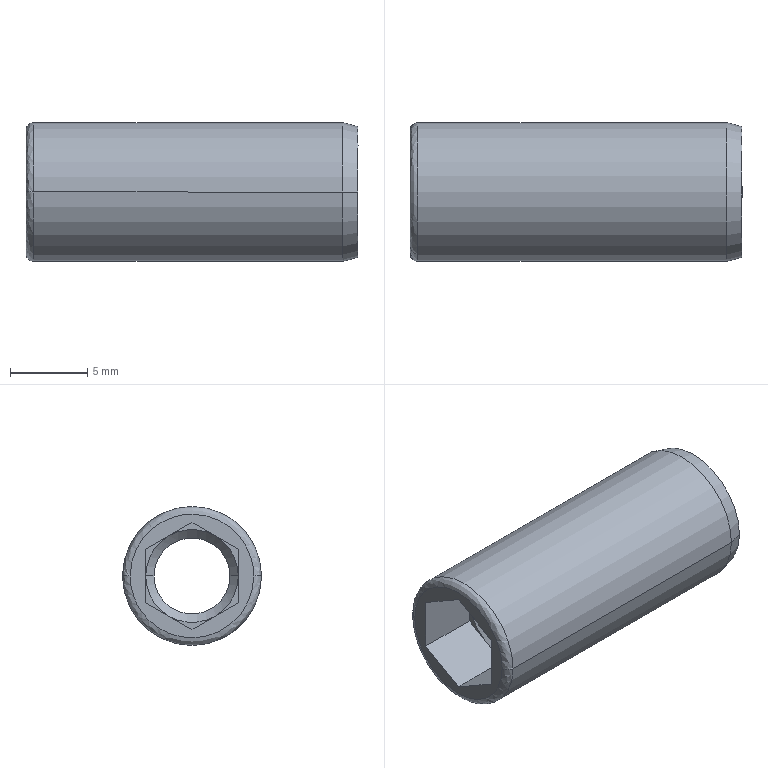Component | SolidWorks | HZ022-SC32x100S-1_HZ022-SC32x100S (10)-1 | 1 solid | 27 faces | box 21.5 x 9 x 9 mm | volume 818 mm3 | plane 15 | cylinder 6 | cone 4 | spline 2 | commonest cylinder face diameters 6.02 x2 9 x2 4.917 x2 | material AL6061
STEP:
#1=CARTESIAN_POINT('',(-11.105,4.179,35.846));
#2=VERTEX_POINT('',#1);
#3=CARTESIAN_POINT('',(-11.105,4.494,35.846));
#4=VERTEX_POINT('',#3);
#5=CARTESIAN_POINT('',(-11.105,4.179,35.846));
#6=CARTESIAN_POINT('',(-11.105,4.179,35.531));
#7=CARTESIAN_POINT('',(-11.105,4.494,35.531));
#8=CARTESIAN_POINT('',(-11.105,4.494,35.846));
#9=(BOUNDED_CURVE()B_SPLINE_CURVE(3,(#5,#6,#7,#8),.UNSPECIFIED.,.F.,.T.)B_SPLINE_CURVE_WITH_KNOTS((4,4),(0.,1.),.UNSPECIFIED.)CURVE()GEOMETRIC_REPRESENTATION_ITEM()RATIONAL_B_SPLINE_CURVE((1.,0.3333,0.3333,1.))REPRESENTATION_ITEM(''));
#10=EDGE_CURVE('',#2,#4,#9,.T.);
#11=ORIENTED_EDGE('',*,*,#10,.T.);
#12=CARTESIAN_POINT('',(-11.085,4.514,35.846));
#13=VERTEX_POINT('',#12);
#14=CARTESIAN_POINT('',(-11.085,4.494,35.846));
#15=DIRECTION('',(-0.,0.,-1.));
#16=DIRECTION('',(0.,1.,0.));
#17=AXIS2_PLACEMENT_3D('',#14,#15,#16);
#18=CIRCLE('',#17,0.01969);
#19=EDGE_CURVE('',#4,#13,#18,.T.);
#20=ORIENTED_EDGE('',*,*,#19,.T.);
#21=CARTESIAN_POINT('',(-11.085,4.16,35.846));
#22=VERTEX_POINT('',#21);
#23=CARTESIAN_POINT('',(-11.085,4.337,35.846));
#24=DIRECTION('',(1.,0.,-0.));
#25=DIRECTION('',(0.,-1.,0.));
#26=AXIS2_PLACEMENT_3D('',#23,#24,#25);
#27=CIRCLE('',#26,0.1772);
#28=EDGE_CURVE('',#22,#13,#27,.T.);
#29=ORIENTED_EDGE('',*,*,#28,.F.);
#30=CARTESIAN_POINT('',(-11.085,4.179,35.846));
#31=DIRECTION('',(0.,-0.,1.));
#32=DIRECTION('',(0.,-1.,0.));
#33=AXIS2_PLACEMENT_3D('',#30,#31,#32);
#34=CIRCLE('',#33,0.01969);
#35=EDGE_CURVE('',#2,#22,#34,.T.);
#36=ORIENTED_EDGE('',*,*,#35,.F.);
#37=EDGE_LOOP('',(#11,#20,#29,#36));
#38=FACE_OUTER_BOUND('',#37,.T.);
#39=CARTESIAN_POINT('',(-11.105,4.494,35.846));
#40=CARTESIAN_POINT('',(-11.105,4.494,35.531));
#41=CARTESIAN_POINT('',(-11.105,4.179,35.531));
#42=CARTESIAN_POINT('',(-11.105,4.179,35.846));
#43=CARTESIAN_POINT('',(-11.105,4.506,35.846));
#44=CARTESIAN_POINT('',(-11.105,4.506,35.508));
#45=CARTESIAN_POINT('',(-11.105,4.168,35.508));
#46=CARTESIAN_POINT('',(-11.105,4.168,35.846));
#47=CARTESIAN_POINT('',(-11.096,4.514,35.846));
#48=CARTESIAN_POINT('',(-11.096,4.514,35.492));
#49=CARTESIAN_POINT('',(-11.096,4.16,35.492));
#50=CARTESIAN_POINT('',(-11.096,4.16,35.846));
#51=CARTESIAN_POINT('',(-11.085,4.514,35.846));
#52=CARTESIAN_POINT('',(-11.085,4.514,35.492));
#53=CARTESIAN_POINT('',(-11.085,4.16,35.492));
#54=CARTESIAN_POINT('',(-11.085,4.16,35.846));
#55=(BOUNDED_SURFACE()B_SPLINE_SURFACE(3,3,((#39,#40,#41,#42),(#43,#44,#45,#46),(#47,#48,#49,#50),(#51,#52,#53,#54)),.UNSPECIFIED.,.F.,.F.,.F.)B_SPLINE_SURFACE_WITH_KNOTS((4,4),(4,4),(0.,1.),(0.,1.),.UNSPECIFIED.)GEOMETRIC_REPRESENTATION_ITEM()RATIONAL_B_SPLINE_SURFACE(((1.,0.3333,0.3333,1.),(0.8047,0.2682,0.2682,0.8047),(0.8047,0.2682,0.2682,0.8047),(1.,0.3333,0.3333,1.)))REPRESENTATION_ITEM('')SURFACE());
#56=ADVANCED_FACE('',(#38),#55,.T.);
#57=CARTESIAN_POINT('',(-10.258,4.218,35.846));
#58=VERTEX_POINT('',#57);
#59=CARTESIAN_POINT('',(-10.258,4.455,35.846));
#60=VERTEX_POINT('',#59);
#61=CARTESIAN_POINT('',(-10.258,4.337,35.846));
#62=DIRECTION('',(-1.,-0.,0.));
#63=DIRECTION('',(0.,-1.,0.));
#64=AXIS2_PLACEMENT_3D('',#61,#62,#63);
#65=CIRCLE('',#64,0.1185);
#66=EDGE_CURVE('',#58,#60,#65,.T.);
#67=ORIENTED_EDGE('',*,*,#66,.F.);
#68=CARTESIAN_POINT('',(-10.612,4.218,35.846));
#69=VERTEX_POINT('',#68);
#70=CARTESIAN_POINT('',(-9.904,4.218,35.846));
#71=DIRECTION('',(-1.,-0.,0.));
#72=VECTOR('',#71,39.37);
#73=LINE('',#70,#72);
#74=EDGE_CURVE('',#58,#69,#73,.T.);
#75=ORIENTED_EDGE('',*,*,#74,.T.);
#76=CARTESIAN_POINT('',(-10.612,4.455,35.846));
#77=VERTEX_POINT('',#76);
#78=CARTESIAN_POINT('',(-10.612,4.337,35.846));
#79=DIRECTION('',(1.,0.,-0.));
#80=DIRECTION('',(0.,-1.,0.));
#81=AXIS2_PLACEMENT_3D('',#78,#79,#80);
#82=CIRCLE('',#81,0.1185);
#83=EDGE_CURVE('',#77,#69,#82,.T.);
#84=ORIENTED_EDGE('',*,*,#83,.F.);
#85=CARTESIAN_POINT('',(-9.904,4.455,35.846));
#86=DIRECTION('',(-1.,-0.,0.));
#87=VECTOR('',#86,39.37);
#88=LINE('',#85,#87);
#89=EDGE_CURVE('',#60,#77,#88,.T.);
#90=ORIENTED_EDGE('',*,*,#89,.F.);
#91=EDGE_LOOP('',(#67,#75,#84,#90));
#92=FACE_OUTER_BOUND('',#91,.T.);
#93=CARTESIAN_POINT('',(-9.904,4.337,35.846));
#94=DIRECTION('',(-1.,-0.,0.));
#95=DIRECTION('',(0.,1.,0.));
#96=AXIS2_PLACEMENT_3D('',#93,#94,#95);
#97=CYLINDRICAL_SURFACE('',#96,0.1185);
#98=ADVANCED_FACE('',(#92),#97,.F.);
#99=ORIENTED_EDGE('',*,*,#28,.T.);
#100=CARTESIAN_POINT('',(-10.297,4.514,35.846));
#101=VERTEX_POINT('',#100);
#102=CARTESIAN_POINT('',(-10.691,4.514,35.846));
#103=DIRECTION('',(1.,0.,-0.));
#104=VECTOR('',#103,39.37);
#105=LINE('',#102,#104);
#106=EDGE_CURVE('',#13,#101,#105,.T.);
#107=ORIENTED_EDGE('',*,*,#106,.T.);
#108=CARTESIAN_POINT('',(-10.297,4.16,35.846));
#109=VERTEX_POINT('',#108);
#110=CARTESIAN_POINT('',(-10.297,4.337,35.846));
#111=DIRECTION('',(-1.,-0.,0.));
#112=DIRECTION('',(0.,-1.,0.));
#113=AXIS2_PLACEMENT_3D('',#110,#111,#112);
#114=CIRCLE('',#113,0.1772);
#115=EDGE_CURVE('',#101,#109,#114,.T.);
#116=ORIENTED_EDGE('',*,*,#115,.T.);
#117=CARTESIAN_POINT('',(-10.691,4.16,35.846));
#118=DIRECTION('',(1.,0.,-0.));
#119=VECTOR('',#118,39.37);
#120=LINE('',#117,#119);
#121=EDGE_CURVE('',#22,#109,#120,.T.);
#122=ORIENTED_EDGE('',*,*,#121,.F.);
#123=EDGE_LOOP('',(#99,#107,#116,#122));
#124=FACE_OUTER_BOUND('',#123,.T.);
#125=CARTESIAN_POINT('',(-10.691,4.337,35.846));
#126=DIRECTION('',(1.,0.,-0.));
#127=DIRECTION('',(0.,-1.,0.));
#128=AXIS2_PLACEMENT_3D('',#125,#126,#127);
#129=CYLINDRICAL_SURFACE('',#128,0.1772);
#130=ADVANCED_FACE('',(#124),#129,.T.);
#131=CARTESIAN_POINT('',(-10.258,4.503,35.846));
#132=VERTEX_POINT('',#131);
#133=CARTESIAN_POINT('',(-10.258,4.17,35.846));
#134=VERTEX_POINT('',#133);
#135=CARTESIAN_POINT('',(-10.258,4.337,35.846));
#136=DIRECTION('',(-1.,-0.,0.));
#137=DIRECTION('',(0.,1.,0.));
#138=AXIS2_PLACEMENT_3D('',#135,#136,#137);
#139=CIRCLE('',#138,0.1666);
#140=EDGE_CURVE('',#132,#134,#139,.T.);
#141=ORIENTED_EDGE('',*,*,#140,.T.);
#142=CARTESIAN_POINT('',(-10.297,4.16,35.846));
#143=DIRECTION('',(-0.9659,-0.2588,0.));
#144=VECTOR('',#143,39.37);
#145=LINE('',#142,#144);
#146=EDGE_CURVE('',#134,#109,#145,.T.);
#147=ORIENTED_EDGE('',*,*,#146,.T.);
#148=ORIENTED_EDGE('',*,*,#115,.F.);
#149=CARTESIAN_POINT('',(-10.297,4.514,35.846));
#150=DIRECTION('',(-0.9659,0.2588,0.));
#151=VECTOR('',#150,39.37);
#152=LINE('',#149,#151);
#153=EDGE_CURVE('',#132,#101,#152,.T.);
#154=ORIENTED_EDGE('',*,*,#153,.F.);
#155=EDGE_LOOP('',(#141,#147,#148,#154));
#156=FACE_OUTER_BOUND('',#155,.T.);
#157=CARTESIAN_POINT('',(-10.297,4.337,35.846));
#158=DIRECTION('',(-1.,-0.,0.));
#159=DIRECTION('',(0.,1.,0.));
#160=AXIS2_PLACEMENT_3D('',#157,#158,#159);
#161=CONICAL_SURFACE('',#160,0.1772,0.2618);
#162=ADVANCED_FACE('',(#156),#161,.T.);
#163=CARTESIAN_POINT('',(-10.926,4.433,35.846));
#164=VERTEX_POINT('',#163);
#165=CARTESIAN_POINT('',(-10.926,4.24,35.846));
#166=VERTEX_POINT('',#165);
#167=CARTESIAN_POINT('',(-10.926,4.337,35.846));
#168=DIRECTION('',(1.,0.,-0.));
#169=DIRECTION('',(0.,-1.,0.));
#170=AXIS2_PLACEMENT_3D('',#167,#168,#169);
#171=CIRCLE('',#170,0.09679);
#172=EDGE_CURVE('',#164,#166,#171,.T.);
#173=ORIENTED_EDGE('',*,*,#172,.T.);
#174=CARTESIAN_POINT('',(-10.947,4.219,35.846));
#175=VERTEX_POINT('',#174);
#176=CARTESIAN_POINT('',(-10.947,4.219,35.846));
#177=DIRECTION('',(-0.7071,-0.7071,0.));
#178=VECTOR('',#177,39.37);
#179=LINE('',#176,#178);
#180=EDGE_CURVE('',#166,#175,#179,.T.);
#181=ORIENTED_EDGE('',*,*,#180,.T.);
#182=CARTESIAN_POINT('',(-10.947,4.278,35.949));
#183=VERTEX_POINT('',#182);
#184=CARTESIAN_POINT('',(-10.947,4.337,35.846));
#185=DIRECTION('',(-1.,-0.,0.));
#186=DIRECTION('',(0.,1.,0.));
#187=AXIS2_PLACEMENT_3D('',#184,#185,#186);
#188=CIRCLE('',#187,0.1181);
#189=EDGE_CURVE('',#175,#183,#188,.T.);
#190=ORIENTED_EDGE('',*,*,#189,.T.);
#191=CARTESIAN_POINT('',(-10.947,4.396,35.949));
#192=VERTEX_POINT('',#191);
#193=CARTESIAN_POINT('',(-10.947,4.337,35.846));
#194=DIRECTION('',(1.,0.,-0.));
#195=DIRECTION('',(0.,1.,0.));
#196=AXIS2_PLACEMENT_3D('',#193,#194,#195);
#197=CIRCLE('',#196,0.1181);
#198=EDGE_CURVE('',#192,#183,#197,.T.);
#199=ORIENTED_EDGE('',*,*,#198,.F.);
#200=CARTESIAN_POINT('',(-10.947,4.455,35.846));
#201=VERTEX_POINT('',#200);
#202=CARTESIAN_POINT('',(-10.947,4.337,35.846));
#203=DIRECTION('',(1.,0.,-0.));
#204=DIRECTION('',(0.,1.,0.));
#205=AXIS2_PLACEMENT_3D('',#202,#203,#204);
#206=CIRCLE('',#205,0.1181);
#207=EDGE_CURVE('',#201,#192,#206,.T.);
#208=ORIENTED_EDGE('',*,*,#207,.F.);
#209=CARTESIAN_POINT('',(-10.947,4.455,35.846));
#210=DIRECTION('',(-0.7071,0.7071,0.));
#211=VECTOR('',#210,39.37);
#212=LINE('',#209,#211);
#213=EDGE_CURVE('',#164,#201,#212,.T.);
#214=ORIENTED_EDGE('',*,*,#213,.F.);
#215=EDGE_LOOP('',(#173,#181,#190,#199,#208,#214));
#216=FACE_OUTER_BOUND('',#215,.T.);
#217=CARTESIAN_POINT('',(-10.947,4.337,35.846));
#218=DIRECTION('',(-1.,-0.,0.));
#219=DIRECTION('',(0.,1.,0.));
#220=AXIS2_PLACEMENT_3D('',#217,#218,#219);
#221=CONICAL_SURFACE('',#220,0.1181,0.7854);
#222=ADVANCED_FACE('',(#216),#221,.F.);
#223=ORIENTED_EDGE('',*,*,#172,.F.);
#224=CARTESIAN_POINT('',(-10.612,4.433,35.846));
#225=VERTEX_POINT('',#224);
#226=CARTESIAN_POINT('',(-10.603,4.433,35.846));
#227=DIRECTION('',(1.,0.,-0.));
#228=VECTOR('',#227,39.37);
#229=LINE('',#226,#228);
#230=EDGE_CURVE('',#164,#225,#229,.T.);
#231=ORIENTED_EDGE('',*,*,#230,.T.);
#232=CARTESIAN_POINT('',(-10.612,4.24,35.846));
#233=VERTEX_POINT('',#232);
#234=CARTESIAN_POINT('',(-10.612,4.337,35.846));
#235=DIRECTION('',(-1.,-0.,0.));
#236=DIRECTION('',(0.,-1.,0.));
#237=AXIS2_PLACEMENT_3D('',#234,#235,#236);
#238=CIRCLE('',#237,0.09679);
#239=EDGE_CURVE('',#233,#225,#238,.T.);
#240=ORIENTED_EDGE('',*,*,#239,.F.);
#241=CARTESIAN_POINT('',(-10.603,4.24,35.846));
#242=DIRECTION('',(1.,0.,-0.));
#243=VECTOR('',#242,39.37);
#244=LINE('',#241,#243);
#245=EDGE_CURVE('',#166,#233,#244,.T.);
#246=ORIENTED_EDGE('',*,*,#245,.F.);
#247=EDGE_LOOP('',(#223,#231,#240,#246));
#248=FACE_OUTER_BOUND('',#247,.T.);
#249=CARTESIAN_POINT('',(-10.603,4.337,35.846));
#250=DIRECTION('',(1.,0.,-0.));
#251=DIRECTION('',(0.,-1.,0.));
#252=AXIS2_PLACEMENT_3D('',#249,#250,#251);
#253=CYLINDRICAL_SURFACE('',#252,0.09679);
#254=ADVANCED_FACE('',(#248),#253,.F.);
#255=ORIENTED_EDGE('',*,*,#230,.F.);
#256=CARTESIAN_POINT('',(-10.926,4.337,35.846));
#257=DIRECTION('',(1.,0.,-0.));
#258=DIRECTION('',(0.,-1.,0.));
#259=AXIS2_PLACEMENT_3D('',#256,#257,#258);
#260=CIRCLE('',#259,0.09679);
#261=EDGE_CURVE('',#166,#164,#260,.T.);
#262=ORIENTED_EDGE('',*,*,#261,.F.);
#263=ORIENTED_EDGE('',*,*,#245,.T.);
#264=CARTESIAN_POINT('',(-10.612,4.337,35.846));
#265=DIRECTION('',(-1.,-0.,0.));
#266=DIRECTION('',(0.,-1.,0.));
#267=AXIS2_PLACEMENT_3D('',#264,#265,#266);
#268=CIRCLE('',#267,0.09679);
#269=EDGE_CURVE('',#225,#233,#268,.T.);
#270=ORIENTED_EDGE('',*,*,#269,.F.);
#271=EDGE_LOOP('',(#255,#262,#263,#270));
#272=FACE_OUTER_BOUND('',#271,.T.);
#273=CARTESIAN_POINT('',(-10.603,4.337,35.846));
#274=DIRECTION('',(1.,0.,-0.));
#275=DIRECTION('',(0.,-1.,0.));
#276=AXIS2_PLACEMENT_3D('',#273,#274,#275);
#277=CYLINDRICAL_SURFACE('',#276,0.09679);
#278=ADVANCED_FACE('',(#272),#277,.F.);
#279=ORIENTED_EDGE('',*,*,#106,.F.);
#280=CARTESIAN_POINT('',(-11.085,4.337,35.846));
#281=DIRECTION('',(1.,0.,-0.));
#282=DIRECTION('',(0.,-1.,0.));
#283=AXIS2_PLACEMENT_3D('',#280,#281,#282);
#284=CIRCLE('',#283,0.1772);
#285=EDGE_CURVE('',#13,#22,#284,.T.);
#286=ORIENTED_EDGE('',*,*,#285,.T.);
#287=ORIENTED_EDGE('',*,*,#121,.T.);
#288=CARTESIAN_POINT('',(-10.297,4.337,35.846));
#289=DIRECTION('',(-1.,-0.,0.));
#290=DIRECTION('',(0.,-1.,0.));
#291=AXIS2_PLACEMENT_3D('',#288,#289,#290);
#292=CIRCLE('',#291,0.1772);
#293=EDGE_CURVE('',#109,#101,#292,.T.);
#294=ORIENTED_EDGE('',*,*,#293,.T.);
#295=EDGE_LOOP('',(#279,#286,#287,#294));
#296=FACE_OUTER_BOUND('',#295,.T.);
#297=CARTESIAN_POINT('',(-10.691,4.337,35.846));
#298=DIRECTION('',(1.,0.,-0.));
#299=DIRECTION('',(0.,-1.,0.));
#300=AXIS2_PLACEMENT_3D('',#297,#298,#299);
#301=CYLINDRICAL_SURFACE('',#300,0.1772);
#302=ADVANCED_FACE('',(#296),#301,.T.);
#303=ORIENTED_EDGE('',*,*,#19,.F.);
#304=CARTESIAN_POINT('',(-11.105,4.337,36.004));
#305=VERTEX_POINT('',#304);
#306=CARTESIAN_POINT('',(-11.105,4.494,35.846));
#307=CARTESIAN_POINT('',(-11.105,4.494,35.939));
#308=CARTESIAN_POINT('',(-11.105,4.429,36.004));
#309=CARTESIAN_POINT('',(-11.105,4.337,36.004));
#310=(BOUNDED_CURVE()B_SPLINE_CURVE(3,(#306,#307,#308,#309),.UNSPECIFIED.,.F.,.T.)B_SPLINE_CURVE_WITH_KNOTS((4,4),(0.,1.),.UNSPECIFIED.)CURVE()GEOMETRIC_REPRESENTATION_ITEM()RATIONAL_B_SPLINE_CURVE((1.,0.8047,0.8047,1.))REPRESENTATION_ITEM(''));
#311=EDGE_CURVE('',#4,#305,#310,.T.);
#312=ORIENTED_EDGE('',*,*,#311,.T.);
#313=CARTESIAN_POINT('',(-11.105,4.337,36.004));
#314=CARTESIAN_POINT('',(-11.105,4.244,36.004));
#315=CARTESIAN_POINT('',(-11.105,4.179,35.939));
#316=CARTESIAN_POINT('',(-11.105,4.179,35.846));
#317=(BOUNDED_CURVE()B_SPLINE_CURVE(3,(#313,#314,#315,#316),.UNSPECIFIED.,.F.,.T.)B_SPLINE_CURVE_WITH_KNOTS((4,4),(0.,1.),.UNSPECIFIED.)CURVE()GEOMETRIC_REPRESENTATION_ITEM()RATIONAL_B_SPLINE_CURVE((1.,0.8047,0.8047,1.))REPRESENTATION_ITEM(''));
#318=EDGE_CURVE('',#305,#2,#317,.T.);
#319=ORIENTED_EDGE('',*,*,#318,.T.);
#320=ORIENTED_EDGE('',*,*,#35,.T.);
#321=ORIENTED_EDGE('',*,*,#285,.F.);
#322=EDGE_LOOP('',(#303,#312,#319,#320,#321));
#323=FACE_OUTER_BOUND('',#322,.T.);
#324=CARTESIAN_POINT('',(-11.105,4.179,35.846));
#325=CARTESIAN_POINT('',(-11.105,4.179,36.161));
#326=CARTESIAN_POINT('',(-11.105,4.494,36.161));
#327=CARTESIAN_POINT('',(-11.105,4.494,35.846));
#328=CARTESIAN_POINT('',(-11.105,4.168,35.846));
#329=CARTESIAN_POINT('',(-11.105,4.168,36.184));
#330=CARTESIAN_POINT('',(-11.105,4.506,36.184));
#331=CARTESIAN_POINT('',(-11.105,4.506,35.846));
#332=CARTESIAN_POINT('',(-11.096,4.16,35.846));
#333=CARTESIAN_POINT('',(-11.096,4.16,36.201));
#334=CARTESIAN_POINT('',(-11.096,4.514,36.201));
#335=CARTESIAN_POINT('',(-11.096,4.514,35.846));
#336=CARTESIAN_POINT('',(-11.085,4.16,35.846));
#337=CARTESIAN_POINT('',(-11.085,4.16,36.201));
#338=CARTESIAN_POINT('',(-11.085,4.514,36.201));
#339=CARTESIAN_POINT('',(-11.085,4.514,35.846));
#340=(BOUNDED_SURFACE()B_SPLINE_SURFACE(3,3,((#324,#325,#326,#327),(#328,#329,#330,#331),(#332,#333,#334,#335),(#336,#337,#338,#339)),.UNSPECIFIED.,.F.,.F.,.T.)B_SPLINE_SURFACE_WITH_KNOTS((4,4),(4,4),(0.,1.),(0.,1.),.UNSPECIFIED.)GEOMETRIC_REPRESENTATION_ITEM()RATIONAL_B_SPLINE_SURFACE(((1.,0.3333,0.3333,1.),(0.8047,0.2682,0.2682,0.8047),(0.8047,0.2682,0.2682,0.8047),(1.,0.3333,0.3333,1.)))REPRESENTATION_ITEM('')SURFACE());
#341=ADVANCED_FACE('',(#323),#340,.T.);
#342=ORIENTED_EDGE('',*,*,#146,.F.);
#343=CARTESIAN_POINT('',(-10.258,4.337,35.846));
#344=DIRECTION('',(-1.,-0.,0.));
#345=DIRECTION('',(0.,1.,0.));
#346=AXIS2_PLACEMENT_3D('',#343,#344,#345);
#347=CIRCLE('',#346,0.1666);
#348=EDGE_CURVE('',#134,#132,#347,.T.);
#349=ORIENTED_EDGE('',*,*,#348,.T.);
#350=ORIENTED_EDGE('',*,*,#153,.T.);
#351=ORIENTED_EDGE('',*,*,#293,.F.);
#352=EDGE_LOOP('',(#342,#349,#350,#351));
#353=FACE_OUTER_BOUND('',#352,.T.);
#354=CARTESIAN_POINT('',(-10.297,4.337,35.846));
#355=DIRECTION('',(-1.,-0.,0.));
#356=DIRECTION('',(0.,1.,0.));
#357=AXIS2_PLACEMENT_3D('',#354,#355,#356);
#358=CONICAL_SURFACE('',#357,0.1772,0.2618);
#359=ADVANCED_FACE('',(#353),#358,.T.);
#360=ORIENTED_EDGE('',*,*,#10,.F.);
#361=ORIENTED_EDGE('',*,*,#318,.F.);
#362=ORIENTED_EDGE('',*,*,#311,.F.);
#363=EDGE_LOOP('',(#360,#361,#362));
#364=FACE_OUTER_BOUND('',#363,.T.);
#365=CARTESIAN_POINT('',(-11.105,4.455,35.778));
#366=VERTEX_POINT('',#365);
#367=CARTESIAN_POINT('',(-11.105,4.455,35.915));
#368=VERTEX_POINT('',#367);
#369=CARTESIAN_POINT('',(-11.105,4.455,35.925));
#370=DIRECTION('',(0.,-0.,1.));
#371=VECTOR('',#370,39.37);
#372=LINE('',#369,#371);
#373=EDGE_CURVE('',#366,#368,#372,.T.);
#374=ORIENTED_EDGE('',*,*,#373,.T.);
#375=CARTESIAN_POINT('',(-11.105,4.337,35.983));
#376=VERTEX_POINT('',#375);
#377=CARTESIAN_POINT('',(-11.105,4.455,35.915));
#378=DIRECTION('',(0.,-0.866,0.5));
#379=VECTOR('',#378,39.37);
#380=LINE('',#377,#379);
#381=EDGE_CURVE('',#368,#376,#380,.T.);
#382=ORIENTED_EDGE('',*,*,#381,.T.);
#383=CARTESIAN_POINT('',(-11.105,4.219,35.915));
#384=VERTEX_POINT('',#383);
#385=CARTESIAN_POINT('',(-11.105,4.337,35.983));
#386=DIRECTION('',(-0.,-0.866,-0.5));
#387=VECTOR('',#386,39.37);
#388=LINE('',#385,#387);
#389=EDGE_CURVE('',#376,#384,#388,.T.);
#390=ORIENTED_EDGE('',*,*,#389,.T.);
#391=CARTESIAN_POINT('',(-11.105,4.219,35.778));
#392=VERTEX_POINT('',#391);
#393=CARTESIAN_POINT('',(-11.105,4.219,35.925));
#394=DIRECTION('',(-0.,0.,-1.));
#395=VECTOR('',#394,39.37);
#396=LINE('',#393,#395);
#397=EDGE_CURVE('',#384,#392,#396,.T.);
#398=ORIENTED_EDGE('',*,*,#397,.T.);
#399=CARTESIAN_POINT('',(-11.105,4.337,35.71));
#400=VERTEX_POINT('',#399);
#401=CARTESIAN_POINT('',(-11.105,4.219,35.778));
#402=DIRECTION('',(-0.,0.866,-0.5));
#403=VECTOR('',#402,39.37);
#404=LINE('',#401,#403);
#405=EDGE_CURVE('',#392,#400,#404,.T.);
#406=ORIENTED_EDGE('',*,*,#405,.T.);
#407=CARTESIAN_POINT('',(-11.105,4.337,35.71));
#408=DIRECTION('',(0.,0.866,0.5));
#409=VECTOR('',#408,39.37);
#410=LINE('',#407,#409);
#411=EDGE_CURVE('',#400,#366,#410,.T.);
#412=ORIENTED_EDGE('',*,*,#411,.T.);
#413=EDGE_LOOP('',(#374,#382,#390,#398,#406,#412));
#414=FACE_BOUND('',#413,.T.);
#415=CARTESIAN_POINT('',(-11.105,4.337,35.925));
#416=DIRECTION('',(-1.,-0.,0.));
#417=DIRECTION('',(-0.,1.,0.));
#418=AXIS2_PLACEMENT_3D('',#415,#416,#417);
#419=PLANE('',#418);
#420=ADVANCED_FACE('',(#364,#414),#419,.T.);
#421=CARTESIAN_POINT('',(-10.258,4.337,35.846));
#422=DIRECTION('',(-1.,-0.,0.));
#423=DIRECTION('',(0.,-1.,-0.));
#424=AXIS2_PLACEMENT_3D('',#421,#422,#423);
#425=CIRCLE('',#424,0.1185);
#426=EDGE_CURVE('',#60,#58,#425,.T.);
#427=ORIENTED_EDGE('',*,*,#426,.T.);
#428=ORIENTED_EDGE('',*,*,#66,.T.);
#429=EDGE_LOOP('',(#427,#428));
#430=FACE_BOUND('',#429,.T.);
#431=ORIENTED_EDGE('',*,*,#140,.F.);
#432=ORIENTED_EDGE('',*,*,#348,.F.);
#433=EDGE_LOOP('',(#431,#432));
#434=FACE_OUTER_BOUND('',#433,.T.);
#435=CARTESIAN_POINT('',(-10.258,4.337,35.93));
#436=DIRECTION('',(1.,0.,-0.));
#437=DIRECTION('',(0.,-1.,-0.));
#438=AXIS2_PLACEMENT_3D('',#435,#436,#437);
#439=PLANE('',#438);
#440=ADVANCED_FACE('',(#430,#434),#439,.T.);
#441=CARTESIAN_POINT('',(-10.947,4.337,35.983));
#442=VERTEX_POINT('',#441);
#443=CARTESIAN_POINT('',(-11.105,4.337,35.983));
#444=DIRECTION('',(1.,0.,-0.));
#445=VECTOR('',#444,39.37);
#446=LINE('',#443,#445);
#447=EDGE_CURVE('',#376,#442,#446,.T.);
#448=ORIENTED_EDGE('',*,*,#447,.F.);
#449=ORIENTED_EDGE('',*,*,#381,.F.);
#450=CARTESIAN_POINT('',(-10.947,4.455,35.915));
#451=VERTEX_POINT('',#450);
#452=CARTESIAN_POINT('',(-11.105,4.455,35.915));
#453=DIRECTION('',(-1.,-0.,0.));
#454=VECTOR('',#453,39.37);
#455=LINE('',#452,#454);
#456=EDGE_CURVE('',#451,#368,#455,.T.);
#457=ORIENTED_EDGE('',*,*,#456,.F.);
#458=CARTESIAN_POINT('',(-10.947,4.455,35.915));
#459=DIRECTION('',(0.,-0.866,0.5));
#460=VECTOR('',#459,39.37);
#461=LINE('',#458,#460);
#462=EDGE_CURVE('',#451,#192,#461,.T.);
#463=ORIENTED_EDGE('',*,*,#462,.T.);
#464=CARTESIAN_POINT('',(-10.947,4.337,35.983));
#465=DIRECTION('',(-0.,0.866,-0.5));
#466=VECTOR('',#465,39.37);
#467=LINE('',#464,#466);
#468=EDGE_CURVE('',#442,#192,#467,.T.);
#469=ORIENTED_EDGE('',*,*,#468,.F.);
#470=EDGE_LOOP('',(#448,#449,#457,#463,#469));
#471=FACE_OUTER_BOUND('',#470,.T.);
#472=CARTESIAN_POINT('',(-11.105,4.337,35.983));
#473=DIRECTION('',(0.,0.5,0.866));
#474=DIRECTION('',(-0.,0.866,-0.5));
#475=AXIS2_PLACEMENT_3D('',#472,#473,#474);
#476=PLANE('',#475);
#477=ADVANCED_FACE('',(#471),#476,.F.);
#478=ORIENTED_EDGE('',*,*,#456,.T.);
#479=ORIENTED_EDGE('',*,*,#373,.F.);
#480=CARTESIAN_POINT('',(-10.947,4.455,35.778));
#481=VERTEX_POINT('',#480);
#482=CARTESIAN_POINT('',(-11.105,4.455,35.778));
#483=DIRECTION('',(-1.,-0.,0.));
#484=VECTOR('',#483,39.37);
#485=LINE('',#482,#484);
#486=EDGE_CURVE('',#481,#366,#485,.T.);
#487=ORIENTED_EDGE('',*,*,#486,.F.);
#488=CARTESIAN_POINT('',(-10.947,4.455,35.846));
#489=DIRECTION('',(0.,-0.,1.));
#490=VECTOR('',#489,39.37);
#491=LINE('',#488,#490);
#492=EDGE_CURVE('',#481,#201,#491,.T.);
#493=ORIENTED_EDGE('',*,*,#492,.T.);
#494=CARTESIAN_POINT('',(-10.947,4.455,35.846));
#495=DIRECTION('',(0.,-0.,1.));
#496=VECTOR('',#495,39.37);
#497=LINE('',#494,#496);
#498=EDGE_CURVE('',#201,#451,#497,.T.);
#499=ORIENTED_EDGE('',*,*,#498,.T.);
#500=EDGE_LOOP('',(#478,#479,#487,#493,#499));
#501=FACE_OUTER_BOUND('',#500,.T.);
#502=CARTESIAN_POINT('',(-11.105,4.455,35.915));
#503=DIRECTION('',(-0.,1.,0.));
#504=DIRECTION('',(1.,0.,-0.));
#505=AXIS2_PLACEMENT_3D('',#502,#503,#504);
#506=PLANE('',#505);
#507=ADVANCED_FACE('',(#501),#506,.F.);
#508=ORIENTED_EDGE('',*,*,#486,.T.);
#509=ORIENTED_EDGE('',*,*,#411,.F.);
#510=CARTESIAN_POINT('',(-10.947,4.337,35.71));
#511=VERTEX_POINT('',#510);
#512=CARTESIAN_POINT('',(-11.105,4.337,35.71));
#513=DIRECTION('',(-1.,-0.,0.));
#514=VECTOR('',#513,39.37);
#515=LINE('',#512,#514);
#516=EDGE_CURVE('',#511,#400,#515,.T.);
#517=ORIENTED_EDGE('',*,*,#516,.F.);
#518=CARTESIAN_POINT('',(-10.947,4.396,35.744));
#519=VERTEX_POINT('',#518);
#520=CARTESIAN_POINT('',(-10.947,4.455,35.778));
#521=DIRECTION('',(-0.,-0.866,-0.5));
#522=VECTOR('',#521,39.37);
#523=LINE('',#520,#522);
#524=EDGE_CURVE('',#519,#511,#523,.T.);
#525=ORIENTED_EDGE('',*,*,#524,.F.);
#526=CARTESIAN_POINT('',(-10.947,4.396,35.744));
#527=DIRECTION('',(0.,0.866,0.5));
#528=VECTOR('',#527,39.37);
#529=LINE('',#526,#528);
#530=EDGE_CURVE('',#519,#481,#529,.T.);
#531=ORIENTED_EDGE('',*,*,#530,.T.);
#532=EDGE_LOOP('',(#508,#509,#517,#525,#531));
#533=FACE_OUTER_BOUND('',#532,.T.);
#534=CARTESIAN_POINT('',(-11.105,4.455,35.778));
#535=DIRECTION('',(-0.,0.5,-0.866));
#536=DIRECTION('',(-0.,-0.866,-0.5));
#537=AXIS2_PLACEMENT_3D('',#534,#535,#536);
#538=PLANE('',#537);
#539=ADVANCED_FACE('',(#533),#538,.F.);
#540=ORIENTED_EDGE('',*,*,#516,.T.);
#541=ORIENTED_EDGE('',*,*,#405,.F.);
#542=CARTESIAN_POINT('',(-10.947,4.219,35.778));
#543=VERTEX_POINT('',#542);
#544=CARTESIAN_POINT('',(-11.105,4.219,35.778));
#545=DIRECTION('',(-1.,-0.,0.));
#546=VECTOR('',#545,39.37);
#547=LINE('',#544,#546);
#548=EDGE_CURVE('',#543,#392,#547,.T.);
#549=ORIENTED_EDGE('',*,*,#548,.F.);
#550=CARTESIAN_POINT('',(-10.947,4.278,35.744));
#551=VERTEX_POINT('',#550);
#552=CARTESIAN_POINT('',(-10.947,4.219,35.778));
#553=DIRECTION('',(-0.,0.866,-0.5));
#554=VECTOR('',#553,39.37);
#555=LINE('',#552,#554);
#556=EDGE_CURVE('',#543,#551,#555,.T.);
#557=ORIENTED_EDGE('',*,*,#556,.T.);
#558=CARTESIAN_POINT('',(-10.947,4.337,35.71));
#559=DIRECTION('',(0.,-0.866,0.5));
#560=VECTOR('',#559,39.37);
#561=LINE('',#558,#560);
#562=EDGE_CURVE('',#511,#551,#561,.T.);
#563=ORIENTED_EDGE('',*,*,#562,.F.);
#564=EDGE_LOOP('',(#540,#541,#549,#557,#563));
#565=FACE_OUTER_BOUND('',#564,.T.);
#566=CARTESIAN_POINT('',(-11.105,4.337,35.71));
#567=DIRECTION('',(-0.,-0.5,-0.866));
#568=DIRECTION('',(0.,-0.866,0.5));
#569=AXIS2_PLACEMENT_3D('',#566,#567,#568);
#570=PLANE('',#569);
#571=ADVANCED_FACE('',(#565),#570,.F.);
#572=ORIENTED_EDGE('',*,*,#548,.T.);
#573=ORIENTED_EDGE('',*,*,#397,.F.);
#574=CARTESIAN_POINT('',(-10.947,4.219,35.915));
#575=VERTEX_POINT('',#574);
#576=CARTESIAN_POINT('',(-11.105,4.219,35.915));
#577=DIRECTION('',(-1.,-0.,0.));
#578=VECTOR('',#577,39.37);
#579=LINE('',#576,#578);
#580=EDGE_CURVE('',#575,#384,#579,.T.);
#581=ORIENTED_EDGE('',*,*,#580,.F.);
#582=CARTESIAN_POINT('',(-10.947,4.219,35.778));
#583=DIRECTION('',(0.,-0.,1.));
#584=VECTOR('',#583,39.37);
#585=LINE('',#582,#584);
#586=EDGE_CURVE('',#175,#575,#585,.T.);
#587=ORIENTED_EDGE('',*,*,#586,.F.);
#588=CARTESIAN_POINT('',(-10.947,4.219,35.846));
#589=DIRECTION('',(-0.,0.,-1.));
#590=VECTOR('',#589,39.37);
#591=LINE('',#588,#590);
#592=EDGE_CURVE('',#175,#543,#591,.T.);
#593=ORIENTED_EDGE('',*,*,#592,.T.);
#594=EDGE_LOOP('',(#572,#573,#581,#587,#593));
#595=FACE_OUTER_BOUND('',#594,.T.);
#596=CARTESIAN_POINT('',(-11.105,4.219,35.778));
#597=DIRECTION('',(0.,-1.,-0.));
#598=DIRECTION('',(-1.,-0.,0.));
#599=AXIS2_PLACEMENT_3D('',#596,#597,#598);
#600=PLANE('',#599);
#601=ADVANCED_FACE('',(#595),#600,.F.);
#602=ORIENTED_EDGE('',*,*,#580,.T.);
#603=ORIENTED_EDGE('',*,*,#389,.F.);
#604=ORIENTED_EDGE('',*,*,#447,.T.);
#605=CARTESIAN_POINT('',(-10.947,4.219,35.915));
#606=DIRECTION('',(0.,0.866,0.5));
#607=VECTOR('',#606,39.37);
#608=LINE('',#605,#607);
#609=EDGE_CURVE('',#183,#442,#608,.T.);
#610=ORIENTED_EDGE('',*,*,#609,.F.);
#611=CARTESIAN_POINT('',(-10.947,4.219,35.915));
#612=DIRECTION('',(0.,0.866,0.5));
#613=VECTOR('',#612,39.37);
#614=LINE('',#611,#613);
#615=EDGE_CURVE('',#575,#183,#614,.T.);
#616=ORIENTED_EDGE('',*,*,#615,.F.);
#617=EDGE_LOOP('',(#602,#603,#604,#610,#616));
#618=FACE_OUTER_BOUND('',#617,.T.);
#619=CARTESIAN_POINT('',(-11.105,4.219,35.915));
#620=DIRECTION('',(0.,-0.5,0.866));
#621=DIRECTION('',(0.,0.866,0.5));
#622=AXIS2_PLACEMENT_3D('',#619,#620,#621);
#623=PLANE('',#622);
#624=ADVANCED_FACE('',(#618),#623,.F.);
#625=ORIENTED_EDGE('',*,*,#198,.T.);
#626=ORIENTED_EDGE('',*,*,#609,.T.);
#627=ORIENTED_EDGE('',*,*,#468,.T.);
#628=EDGE_LOOP('',(#625,#626,#627));
#629=FACE_OUTER_BOUND('',#628,.T.);
#630=CARTESIAN_POINT('',(-10.947,4.337,35.846));
#631=DIRECTION('',(1.,0.,-0.));
#632=DIRECTION('',(0.,-1.,-0.));
#633=AXIS2_PLACEMENT_3D('',#630,#631,#632);
#634=PLANE('',#633);
#635=ADVANCED_FACE('',(#629),#634,.F.);
#636=CARTESIAN_POINT('',(-10.947,4.337,35.846));
#637=DIRECTION('',(1.,0.,-0.));
#638=DIRECTION('',(0.,1.,-0.));
#639=AXIS2_PLACEMENT_3D('',#636,#637,#638);
#640=CIRCLE('',#639,0.1181);
#641=EDGE_CURVE('',#551,#519,#640,.T.);
#642=ORIENTED_EDGE('',*,*,#641,.T.);
#643=ORIENTED_EDGE('',*,*,#524,.T.);
#644=ORIENTED_EDGE('',*,*,#562,.T.);
#645=EDGE_LOOP('',(#642,#643,#644));
#646=FACE_OUTER_BOUND('',#645,.T.);
#647=CARTESIAN_POINT('',(-10.947,4.337,35.846));
#648=DIRECTION('',(1.,0.,-0.));
#649=DIRECTION('',(0.,-1.,-0.));
#650=AXIS2_PLACEMENT_3D('',#647,#648,#649);
#651=PLANE('',#650);
#652=ADVANCED_FACE('',(#646),#651,.F.);
#653=ORIENTED_EDGE('',*,*,#586,.T.);
#654=ORIENTED_EDGE('',*,*,#615,.T.);
#655=ORIENTED_EDGE('',*,*,#189,.F.);
#656=EDGE_LOOP('',(#653,#654,#655));
#657=FACE_OUTER_BOUND('',#656,.T.);
#658=CARTESIAN_POINT('',(-10.947,4.337,35.846));
#659=DIRECTION('',(1.,0.,-0.));
#660=DIRECTION('',(0.,-1.,-0.));
#661=AXIS2_PLACEMENT_3D('',#658,#659,#660);
#662=PLANE('',#661);
#663=ADVANCED_FACE('',(#657),#662,.F.);
#664=ORIENTED_EDGE('',*,*,#180,.F.);
#665=ORIENTED_EDGE('',*,*,#261,.T.);
#666=ORIENTED_EDGE('',*,*,#213,.T.);
#667=CARTESIAN_POINT('',(-10.947,4.337,35.846));
#668=DIRECTION('',(1.,0.,-0.));
#669=DIRECTION('',(0.,1.,0.));
#670=AXIS2_PLACEMENT_3D('',#667,#668,#669);
#671=CIRCLE('',#670,0.1181);
#672=EDGE_CURVE('',#519,#201,#671,.T.);
#673=ORIENTED_EDGE('',*,*,#672,.F.);
#674=ORIENTED_EDGE('',*,*,#641,.F.);
#675=CARTESIAN_POINT('',(-10.947,4.337,35.846));
#676=DIRECTION('',(1.,0.,-0.));
#677=DIRECTION('',(0.,1.,0.));
#678=AXIS2_PLACEMENT_3D('',#675,#676,#677);
#679=CIRCLE('',#678,0.1181);
#680=EDGE_CURVE('',#175,#551,#679,.T.);
#681=ORIENTED_EDGE('',*,*,#680,.F.);
#682=EDGE_LOOP('',(#664,#665,#666,#673,#674,#681));
#683=FACE_OUTER_BOUND('',#682,.T.);
#684=CARTESIAN_POINT('',(-10.947,4.337,35.846));
#685=DIRECTION('',(-1.,-0.,0.));
#686=DIRECTION('',(0.,1.,0.));
#687=AXIS2_PLACEMENT_3D('',#684,#685,#686);
#688=CONICAL_SURFACE('',#687,0.1181,0.7854);
#689=ADVANCED_FACE('',(#683),#688,.F.);
#690=ORIENTED_EDGE('',*,*,#556,.F.);
#691=ORIENTED_EDGE('',*,*,#592,.F.);
#692=ORIENTED_EDGE('',*,*,#680,.T.);
#693=EDGE_LOOP('',(#690,#691,#692));
#694=FACE_OUTER_BOUND('',#693,.T.);
#695=CARTESIAN_POINT('',(-10.947,4.337,35.846));
#696=DIRECTION('',(1.,0.,-0.));
#697=DIRECTION('',(0.,-1.,-0.));
#698=AXIS2_PLACEMENT_3D('',#695,#696,#697);
#699=PLANE('',#698);
#700=ADVANCED_FACE('',(#694),#699,.F.);
#701=ORIENTED_EDGE('',*,*,#462,.F.);
#702=ORIENTED_EDGE('',*,*,#498,.F.);
#703=ORIENTED_EDGE('',*,*,#207,.T.);
#704=EDGE_LOOP('',(#701,#702,#703));
#705=FACE_OUTER_BOUND('',#704,.T.);
#706=CARTESIAN_POINT('',(-10.947,4.337,35.846));
#707=DIRECTION('',(1.,0.,-0.));
#708=DIRECTION('',(0.,-1.,-0.));
#709=AXIS2_PLACEMENT_3D('',#706,#707,#708);
#710=PLANE('',#709);
#711=ADVANCED_FACE('',(#705),#710,.F.);
#712=ORIENTED_EDGE('',*,*,#492,.F.);
#713=ORIENTED_EDGE('',*,*,#530,.F.);
#714=ORIENTED_EDGE('',*,*,#672,.T.);
#715=EDGE_LOOP('',(#712,#713,#714));
#716=FACE_OUTER_BOUND('',#715,.T.);
#717=CARTESIAN_POINT('',(-10.947,4.337,35.846));
#718=DIRECTION('',(1.,0.,-0.));
#719=DIRECTION('',(0.,-1.,-0.));
#720=AXIS2_PLACEMENT_3D('',#717,#718,#719);
#721=PLANE('',#720);
#722=ADVANCED_FACE('',(#716),#721,.F.);
#723=ORIENTED_EDGE('',*,*,#83,.T.);
#724=CARTESIAN_POINT('',(-10.612,4.337,35.846));
#725=DIRECTION('',(1.,0.,-0.));
#726=DIRECTION('',(0.,-1.,0.));
#727=AXIS2_PLACEMENT_3D('',#724,#725,#726);
#728=CIRCLE('',#727,0.1185);
#729=EDGE_CURVE('',#69,#77,#728,.T.);
#730=ORIENTED_EDGE('',*,*,#729,.T.);
#731=EDGE_LOOP('',(#723,#730));
#732=FACE_OUTER_BOUND('',#731,.T.);
#733=ORIENTED_EDGE('',*,*,#239,.T.);
#734=ORIENTED_EDGE('',*,*,#269,.T.);
#735=EDGE_LOOP('',(#733,#734));
#736=FACE_BOUND('',#735,.T.);
#737=CARTESIAN_POINT('',(-10.612,4.337,35.846));
#738=DIRECTION('',(1.,0.,-0.));
#739=DIRECTION('',(0.,-1.,-0.));
#740=AXIS2_PLACEMENT_3D('',#737,#738,#739);
#741=PLANE('',#740);
#742=ADVANCED_FACE('',(#732,#736),#741,.T.);
#743=ORIENTED_EDGE('',*,*,#74,.F.);
#744=ORIENTED_EDGE('',*,*,#426,.F.);
#745=ORIENTED_EDGE('',*,*,#89,.T.);
#746=ORIENTED_EDGE('',*,*,#729,.F.);
#747=EDGE_LOOP('',(#743,#744,#745,#746));
#748=FACE_OUTER_BOUND('',#747,.T.);
#749=CARTESIAN_POINT('',(-9.904,4.337,35.846));
#750=DIRECTION('',(-1.,-0.,0.));
#751=DIRECTION('',(0.,1.,0.));
#752=AXIS2_PLACEMENT_3D('',#749,#750,#751);
#753=CYLINDRICAL_SURFACE('',#752,0.1185);
#754=ADVANCED_FACE('',(#748),#753,.F.);
#755=CLOSED_SHELL('',(#56,#98,#130,#162,#222,#254,#278,#302,#341,#359,#420,#440,#477,#507,#539,#571,#601,#624,#635,#652,#663,#689,#700,#711,#722,#742,#754));
#756=MANIFOLD_SOLID_BREP('',#755);
#757=CARTESIAN_POINT('',(0.,0.,0.));
#758=DIRECTION('',(0.,0.,1.));
#759=DIRECTION('',(1.,0.,0.));
#760=AXIS2_PLACEMENT_3D('',#757,#758,#759);
#761=(LENGTH_UNIT()NAMED_UNIT(*)SI_UNIT($,.METRE.));
#762=LENGTH_MEASURE_WITH_UNIT(LENGTH_MEASURE(0.0254),#761);
#763=DIMENSIONAL_EXPONENTS(1.,0.,0.,0.,0.,0.,0.);
#764=(CONVERSION_BASED_UNIT('',#762)LENGTH_UNIT()NAMED_UNIT(#763));
#765=UNCERTAINTY_MEASURE_WITH_UNIT(LENGTH_MEASURE(0.00001),#764,'','');
#766=(NAMED_UNIT(*)PLANE_ANGLE_UNIT()SI_UNIT($,.RADIAN.));
#767=(NAMED_UNIT(*)SI_UNIT($,.STERADIAN.)SOLID_ANGLE_UNIT());
#768=(GEOMETRIC_REPRESENTATION_CONTEXT(3)GLOBAL_UNCERTAINTY_ASSIGNED_CONTEXT((#765))GLOBAL_UNIT_ASSIGNED_CONTEXT((#764,#766,#767))REPRESENTATION_CONTEXT('',''));
#769=ADVANCED_BREP_SHAPE_REPRESENTATION('',(#756,#760),#768);
#770=COLOUR_RGB('',0.7922,0.8196,0.9333);
#771=FILL_AREA_STYLE_COLOUR('',#770);
#772=FILL_AREA_STYLE('',(#771));
#773=SURFACE_STYLE_FILL_AREA(#772);
#774=SURFACE_SIDE_STYLE('',(#773));
#775=SURFACE_STYLE_USAGE(.BOTH.,#774);
#776=PRESENTATION_STYLE_ASSIGNMENT((#775));
#777=STYLED_ITEM('',(#776),#756);
#778=(LENGTH_UNIT()NAMED_UNIT(*)SI_UNIT($,.METRE.));
#779=LENGTH_MEASURE_WITH_UNIT(LENGTH_MEASURE(0.0254),#778);
#780=DIMENSIONAL_EXPONENTS(1.,0.,0.,0.,0.,0.,0.);
#781=(CONVERSION_BASED_UNIT('',#779)LENGTH_UNIT()NAMED_UNIT(#780));
#782=UNCERTAINTY_MEASURE_WITH_UNIT(LENGTH_MEASURE(0.00001),#781,'','');
#783=(NAMED_UNIT(*)PLANE_ANGLE_UNIT()SI_UNIT($,.RADIAN.));
#784=(NAMED_UNIT(*)SI_UNIT($,.STERADIAN.)SOLID_ANGLE_UNIT());
#785=(GEOMETRIC_REPRESENTATION_CONTEXT(3)GLOBAL_UNCERTAINTY_ASSIGNED_CONTEXT((#782))GLOBAL_UNIT_ASSIGNED_CONTEXT((#781,#783,#784))REPRESENTATION_CONTEXT('',''));
#786=MECHANICAL_DESIGN_GEOMETRIC_PRESENTATION_REPRESENTATION('',(#777),#785);
#787=PRESENTATION_LAYER_ASSIGNMENT('','',(#777));